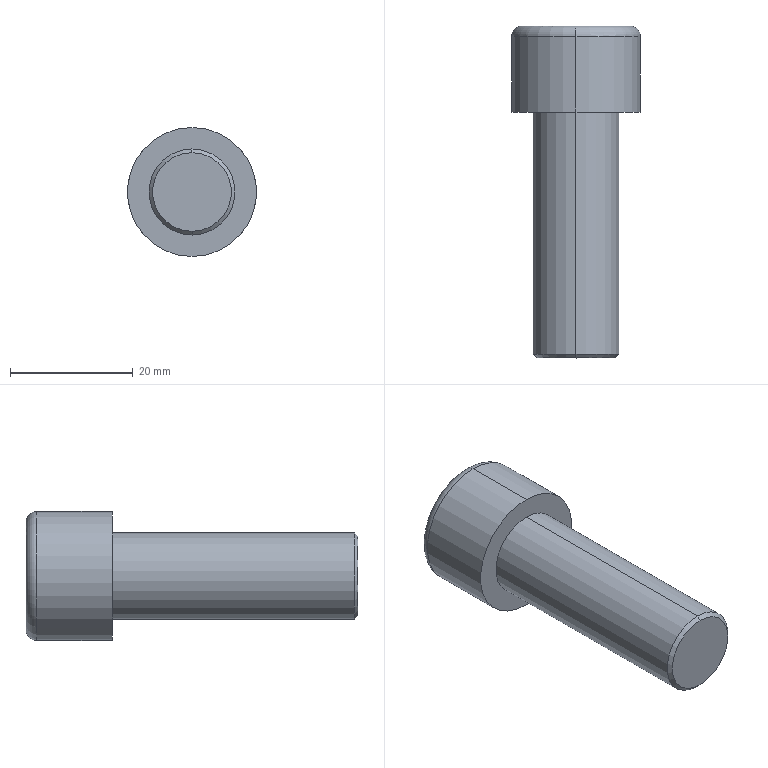Component | SolidWorks | hexagon socket head cap screws gb-100 | 1 solid | 25 faces | box 21 x 54 x 21 mm | volume 9954 mm3 | plane 15 | cone 4 | cylinder 4 | torus 2 | commonest cylinder face diameters 14 x2 21 x2
build123d program:
from build123d import *

# Parameters (mm, degrees)
SKETCH1_R           = 10.5
BASEHEAD_DEPTH      = 14
SKETCH2_R           = 7
BASEBODY_DEPTH      = 40
HEXAGONSOCKET_DEPTH = 7
TOPFILLET_R         = 1.75
CHAMFER1_SIZE       = 0.6


with BuildPart() as part:
    # Sketch1 → BaseHead (new body)
    with BuildSketch(Plane(origin=(0, 0, 0), x_dir=(0, 0, -1), z_dir=(1, 0, 0))):
        Circle(SKETCH1_R)
    extrude(amount=BASEHEAD_DEPTH)

    # Sketch2 → BaseBody (add)
    with BuildSketch(Plane(origin=(14, 0, 0), x_dir=(0, 0, -1), z_dir=(1, 0, 0))):
        Circle(SKETCH2_R)
    extrude(amount=BASEBODY_DEPTH)

    # Sketch3 → HexagonSocket (cut)
    with BuildSketch(Plane(origin=(0, 0, 0), x_dir=(0, 0, -1), z_dir=(1, 0, 0))):
        Polygon((6.928, 0), (3.464, 6), (-3.464, 6), (-6.928, 0), (-3.464, -6), (3.464, -6), align=None)
    extrude(amount=HEXAGONSOCKET_DEPTH, mode=Mode.SUBTRACT)

    # Sketch4 → Cut-Revolve1 (revolve, cut)
    with BuildSketch(Plane(origin=(-4.196, 0.75, 0), x_dir=(-1, 0, 0), z_dir=(0, 0, 1)), mode=Mode.PRIVATE) as cut_revolve1_sk:
        Polygon((-11.196, 6.75), (-14.66, 0.75), (-11.196, 0.75), align=None)
    revolve(cut_revolve1_sk.sketch.rotate(Axis((0.839, 0, 0), (-1, 0, 0)), 90), axis=Axis((0.839, 0, 0), (-1, 0, 0)), mode=Mode.SUBTRACT)

    # TopFillet
    topfillet_edges = [part.edges().sort_by_distance(p)[0] for p in [
        (0, 0, 10.5),
    ]]
    fillet(topfillet_edges, radius=TOPFILLET_R)

    # Chamfer1
    chamfer1_edges = [part.edges().sort_by_distance(p)[0] for p in [
        (54, 0, 7),
    ]]
    chamfer(chamfer1_edges, length=CHAMFER1_SIZE)


solid = part.part

# Placed as in the assembly
solid = solid.moved(Location((34.577, 214.019, 538.347), (0, 0, -90)))
STEP:
#1=COLOUR_RGB('',0.7922,0.8196,0.9333);
#2=FILL_AREA_STYLE_COLOUR('',#1);
#3=FILL_AREA_STYLE('',(#2));
#4=SURFACE_STYLE_FILL_AREA(#3);
#5=SURFACE_SIDE_STYLE('',(#4));
#6=SURFACE_STYLE_USAGE(.BOTH.,#5);
#7=PRESENTATION_STYLE_ASSIGNMENT((#6));
#8=CARTESIAN_POINT('',(1.361,6.3,21.447));
#9=VERTEX_POINT('',#8);
#10=CARTESIAN_POINT('',(1.361,6.3,20.943));
#11=VERTEX_POINT('',#10);
#12=CARTESIAN_POINT('',(1.361,6.3,21.195));
#13=DIRECTION('',(0.,-1.,0.));
#14=DIRECTION('',(-0.,0.,1.));
#15=AXIS2_PLACEMENT_3D('',#12,#13,#14);
#16=CIRCLE('',#15,0.252);
#17=EDGE_CURVE('',#9,#11,#16,.T.);
#18=ORIENTED_EDGE('',*,*,#17,.F.);
#19=CARTESIAN_POINT('',(1.361,6.324,21.47));
#20=VERTEX_POINT('',#19);
#21=CARTESIAN_POINT('',(1.361,6.3,21.447));
#22=DIRECTION('',(-0.,0.7071,0.7071));
#23=VECTOR('',#22,39.37);
#24=LINE('',#21,#23);
#25=EDGE_CURVE('',#9,#20,#24,.T.);
#26=ORIENTED_EDGE('',*,*,#25,.T.);
#27=CARTESIAN_POINT('',(1.361,6.324,20.919));
#28=VERTEX_POINT('',#27);
#29=CARTESIAN_POINT('',(1.361,6.324,21.195));
#30=DIRECTION('',(0.,1.,0.));
#31=DIRECTION('',(-0.,0.,1.));
#32=AXIS2_PLACEMENT_3D('',#29,#30,#31);
#33=CIRCLE('',#32,0.2756);
#34=EDGE_CURVE('',#28,#20,#33,.T.);
#35=ORIENTED_EDGE('',*,*,#34,.F.);
#36=CARTESIAN_POINT('',(1.361,6.3,20.943));
#37=DIRECTION('',(0.,0.7071,-0.7071));
#38=VECTOR('',#37,39.37);
#39=LINE('',#36,#38);
#40=EDGE_CURVE('',#11,#28,#39,.T.);
#41=ORIENTED_EDGE('',*,*,#40,.F.);
#42=EDGE_LOOP('',(#18,#26,#35,#41));
#43=FACE_OUTER_BOUND('',#42,.T.);
#44=CARTESIAN_POINT('',(1.361,6.3,21.195));
#45=DIRECTION('',(0.,1.,0.));
#46=DIRECTION('',(0.,0.,-1.));
#47=AXIS2_PLACEMENT_3D('',#44,#45,#46);
#48=CONICAL_SURFACE('',#47,0.252,0.7854);
#49=ADVANCED_FACE('',(#43),#48,.T.);
#50=CARTESIAN_POINT('',(1.361,8.426,20.85));
#51=VERTEX_POINT('',#50);
#52=CARTESIAN_POINT('',(1.361,8.426,21.539));
#53=VERTEX_POINT('',#52);
#54=CARTESIAN_POINT('',(1.361,8.426,21.195));
#55=DIRECTION('',(0.,1.,0.));
#56=DIRECTION('',(-0.,0.,1.));
#57=AXIS2_PLACEMENT_3D('',#54,#55,#56);
#58=CIRCLE('',#57,0.3445);
#59=EDGE_CURVE('',#51,#53,#58,.T.);
#60=ORIENTED_EDGE('',*,*,#59,.F.);
#61=CARTESIAN_POINT('',(1.361,8.357,20.781));
#62=VERTEX_POINT('',#61);
#63=CARTESIAN_POINT('',(1.361,8.357,20.85));
#64=DIRECTION('',(-1.,0.,-0.));
#65=DIRECTION('',(-0.,0.,1.));
#66=AXIS2_PLACEMENT_3D('',#63,#64,#65);
#67=CIRCLE('',#66,0.0689);
#68=EDGE_CURVE('',#51,#62,#67,.T.);
#69=ORIENTED_EDGE('',*,*,#68,.T.);
#70=CARTESIAN_POINT('',(1.361,8.357,21.608));
#71=VERTEX_POINT('',#70);
#72=CARTESIAN_POINT('',(1.361,8.357,21.195));
#73=DIRECTION('',(0.,-1.,0.));
#74=DIRECTION('',(-0.,0.,1.));
#75=AXIS2_PLACEMENT_3D('',#72,#73,#74);
#76=CIRCLE('',#75,0.4134);
#77=EDGE_CURVE('',#71,#62,#76,.T.);
#78=ORIENTED_EDGE('',*,*,#77,.F.);
#79=CARTESIAN_POINT('',(1.361,8.357,21.539));
#80=DIRECTION('',(1.,0.,0.));
#81=DIRECTION('',(0.,0.,-1.));
#82=AXIS2_PLACEMENT_3D('',#79,#80,#81);
#83=CIRCLE('',#82,0.0689);
#84=EDGE_CURVE('',#53,#71,#83,.T.);
#85=ORIENTED_EDGE('',*,*,#84,.F.);
#86=EDGE_LOOP('',(#60,#69,#78,#85));
#87=FACE_OUTER_BOUND('',#86,.T.);
#88=CARTESIAN_POINT('',(1.361,8.357,21.195));
#89=DIRECTION('',(0.,-1.,0.));
#90=DIRECTION('',(-0.,0.,1.));
#91=AXIS2_PLACEMENT_3D('',#88,#89,#90);
#92=TOROIDAL_SURFACE('',#91,0.3445,0.0689);
#93=ADVANCED_FACE('',(#87),#92,.T.);
#94=CARTESIAN_POINT('',(1.361,8.014,21.195));
#95=VERTEX_POINT('',#94);
#96=CARTESIAN_POINT('',(1.361,8.15,20.959));
#97=VERTEX_POINT('',#96);
#98=CARTESIAN_POINT('',(1.361,8.15,20.959));
#99=DIRECTION('',(0.,0.5,-0.866));
#100=VECTOR('',#99,39.37);
#101=LINE('',#98,#100);
#102=EDGE_CURVE('',#95,#97,#101,.T.);
#103=ORIENTED_EDGE('',*,*,#102,.F.);
#104=CARTESIAN_POINT('',(1.361,8.15,21.431));
#105=VERTEX_POINT('',#104);
#106=CARTESIAN_POINT('',(1.361,8.15,21.431));
#107=DIRECTION('',(-0.,0.5,0.866));
#108=VECTOR('',#107,39.37);
#109=LINE('',#106,#108);
#110=EDGE_CURVE('',#95,#105,#109,.T.);
#111=ORIENTED_EDGE('',*,*,#110,.T.);
#112=CARTESIAN_POINT('',(1.479,8.15,21.399));
#113=VERTEX_POINT('',#112);
#114=CARTESIAN_POINT('',(1.361,8.15,21.195));
#115=DIRECTION('',(0.,-1.,0.));
#116=DIRECTION('',(0.,0.,-1.));
#117=AXIS2_PLACEMENT_3D('',#114,#115,#116);
#118=CIRCLE('',#117,0.2362);
#119=EDGE_CURVE('',#113,#105,#118,.T.);
#120=ORIENTED_EDGE('',*,*,#119,.F.);
#121=CARTESIAN_POINT('',(1.598,8.15,21.195));
#122=VERTEX_POINT('',#121);
#123=CARTESIAN_POINT('',(1.361,8.15,21.195));
#124=DIRECTION('',(0.,-1.,0.));
#125=DIRECTION('',(0.,0.,-1.));
#126=AXIS2_PLACEMENT_3D('',#123,#124,#125);
#127=CIRCLE('',#126,0.2362);
#128=EDGE_CURVE('',#122,#113,#127,.T.);
#129=ORIENTED_EDGE('',*,*,#128,.F.);
#130=CARTESIAN_POINT('',(1.479,8.15,20.99));
#131=VERTEX_POINT('',#130);
#132=CARTESIAN_POINT('',(1.361,8.15,21.195));
#133=DIRECTION('',(0.,-1.,0.));
#134=DIRECTION('',(0.,0.,-1.));
#135=AXIS2_PLACEMENT_3D('',#132,#133,#134);
#136=CIRCLE('',#135,0.2362);
#137=EDGE_CURVE('',#131,#122,#136,.T.);
#138=ORIENTED_EDGE('',*,*,#137,.F.);
#139=CARTESIAN_POINT('',(1.361,8.15,21.195));
#140=DIRECTION('',(0.,-1.,0.));
#141=DIRECTION('',(0.,0.,-1.));
#142=AXIS2_PLACEMENT_3D('',#139,#140,#141);
#143=CIRCLE('',#142,0.2362);
#144=EDGE_CURVE('',#97,#131,#143,.T.);
#145=ORIENTED_EDGE('',*,*,#144,.F.);
#146=EDGE_LOOP('',(#103,#111,#120,#129,#138,#145));
#147=FACE_OUTER_BOUND('',#146,.T.);
#148=CARTESIAN_POINT('',(1.361,8.15,21.195));
#149=DIRECTION('',(0.,1.,0.));
#150=DIRECTION('',(0.,0.,-1.));
#151=AXIS2_PLACEMENT_3D('',#148,#149,#150);
#152=CONICAL_SURFACE('',#151,0.2362,1.047);
#153=ADVANCED_FACE('',(#147),#152,.F.);
#154=ORIENTED_EDGE('',*,*,#34,.T.);
#155=CARTESIAN_POINT('',(1.361,7.875,21.47));
#156=VERTEX_POINT('',#155);
#157=CARTESIAN_POINT('',(1.361,6.3,21.47));
#158=DIRECTION('',(0.,1.,0.));
#159=VECTOR('',#158,39.37);
#160=LINE('',#157,#159);
#161=EDGE_CURVE('',#20,#156,#160,.T.);
#162=ORIENTED_EDGE('',*,*,#161,.T.);
#163=CARTESIAN_POINT('',(1.361,7.875,20.919));
#164=VERTEX_POINT('',#163);
#165=CARTESIAN_POINT('',(1.361,7.875,21.195));
#166=DIRECTION('',(0.,-1.,0.));
#167=DIRECTION('',(-0.,0.,1.));
#168=AXIS2_PLACEMENT_3D('',#165,#166,#167);
#169=CIRCLE('',#168,0.2756);
#170=EDGE_CURVE('',#156,#164,#169,.T.);
#171=ORIENTED_EDGE('',*,*,#170,.T.);
#172=CARTESIAN_POINT('',(1.361,6.3,20.919));
#173=DIRECTION('',(0.,1.,0.));
#174=VECTOR('',#173,39.37);
#175=LINE('',#172,#174);
#176=EDGE_CURVE('',#28,#164,#175,.T.);
#177=ORIENTED_EDGE('',*,*,#176,.F.);
#178=EDGE_LOOP('',(#154,#162,#171,#177));
#179=FACE_OUTER_BOUND('',#178,.T.);
#180=CARTESIAN_POINT('',(1.361,6.3,21.195));
#181=DIRECTION('',(0.,1.,0.));
#182=DIRECTION('',(0.,0.,-1.));
#183=AXIS2_PLACEMENT_3D('',#180,#181,#182);
#184=CYLINDRICAL_SURFACE('',#183,0.2756);
#185=ADVANCED_FACE('',(#179),#184,.T.);
#186=CARTESIAN_POINT('',(1.361,7.875,21.608));
#187=VERTEX_POINT('',#186);
#188=CARTESIAN_POINT('',(1.361,7.875,20.781));
#189=VERTEX_POINT('',#188);
#190=CARTESIAN_POINT('',(1.361,7.875,21.195));
#191=DIRECTION('',(0.,-1.,0.));
#192=DIRECTION('',(-0.,0.,1.));
#193=AXIS2_PLACEMENT_3D('',#190,#191,#192);
#194=CIRCLE('',#193,0.4134);
#195=EDGE_CURVE('',#187,#189,#194,.T.);
#196=ORIENTED_EDGE('',*,*,#195,.F.);
#197=CARTESIAN_POINT('',(1.361,7.875,21.608));
#198=DIRECTION('',(0.,1.,0.));
#199=VECTOR('',#198,39.37);
#200=LINE('',#197,#199);
#201=EDGE_CURVE('',#187,#71,#200,.T.);
#202=ORIENTED_EDGE('',*,*,#201,.T.);
#203=ORIENTED_EDGE('',*,*,#77,.T.);
#204=CARTESIAN_POINT('',(1.361,7.875,20.781));
#205=DIRECTION('',(0.,1.,0.));
#206=VECTOR('',#205,39.37);
#207=LINE('',#204,#206);
#208=EDGE_CURVE('',#189,#62,#207,.T.);
#209=ORIENTED_EDGE('',*,*,#208,.F.);
#210=EDGE_LOOP('',(#196,#202,#203,#209));
#211=FACE_OUTER_BOUND('',#210,.T.);
#212=CARTESIAN_POINT('',(1.361,7.875,21.195));
#213=DIRECTION('',(0.,1.,0.));
#214=DIRECTION('',(0.,0.,-1.));
#215=AXIS2_PLACEMENT_3D('',#212,#213,#214);
#216=CYLINDRICAL_SURFACE('',#215,0.4134);
#217=ADVANCED_FACE('',(#211),#216,.T.);
#218=CARTESIAN_POINT('',(1.598,8.15,21.058));
#219=VERTEX_POINT('',#218);
#220=CARTESIAN_POINT('',(1.361,8.15,20.922));
#221=DIRECTION('',(0.866,0.,0.5));
#222=VECTOR('',#221,39.37);
#223=LINE('',#220,#222);
#224=EDGE_CURVE('',#131,#219,#223,.T.);
#225=ORIENTED_EDGE('',*,*,#224,.F.);
#226=ORIENTED_EDGE('',*,*,#137,.T.);
#227=CARTESIAN_POINT('',(1.598,8.15,21.058));
#228=DIRECTION('',(-0.,0.,1.));
#229=VECTOR('',#228,39.37);
#230=LINE('',#227,#229);
#231=EDGE_CURVE('',#219,#122,#230,.T.);
#232=ORIENTED_EDGE('',*,*,#231,.F.);
#233=EDGE_LOOP('',(#225,#226,#232));
#234=FACE_OUTER_BOUND('',#233,.T.);
#235=CARTESIAN_POINT('',(1.834,8.15,21.195));
#236=DIRECTION('',(0.,1.,0.));
#237=DIRECTION('',(0.,0.,-1.));
#238=AXIS2_PLACEMENT_3D('',#235,#236,#237);
#239=PLANE('',#238);
#240=ADVANCED_FACE('',(#234),#239,.T.);
#241=CARTESIAN_POINT('',(1.598,8.15,21.331));
#242=VERTEX_POINT('',#241);
#243=CARTESIAN_POINT('',(1.598,8.15,21.058));
#244=DIRECTION('',(-0.,0.,1.));
#245=VECTOR('',#244,39.37);
#246=LINE('',#243,#245);
#247=EDGE_CURVE('',#122,#242,#246,.T.);
#248=ORIENTED_EDGE('',*,*,#247,.F.);
#249=ORIENTED_EDGE('',*,*,#128,.T.);
#250=CARTESIAN_POINT('',(1.598,8.15,21.331));
#251=DIRECTION('',(-0.866,0.,0.5));
#252=VECTOR('',#251,39.37);
#253=LINE('',#250,#252);
#254=EDGE_CURVE('',#242,#113,#253,.T.);
#255=ORIENTED_EDGE('',*,*,#254,.F.);
#256=EDGE_LOOP('',(#248,#249,#255));
#257=FACE_OUTER_BOUND('',#256,.T.);
#258=CARTESIAN_POINT('',(1.834,8.15,21.195));
#259=DIRECTION('',(0.,1.,0.));
#260=DIRECTION('',(0.,0.,-1.));
#261=AXIS2_PLACEMENT_3D('',#258,#259,#260);
#262=PLANE('',#261);
#263=ADVANCED_FACE('',(#257),#262,.T.);
#264=CARTESIAN_POINT('',(1.361,8.15,21.468));
#265=VERTEX_POINT('',#264);
#266=CARTESIAN_POINT('',(1.598,8.15,21.331));
#267=DIRECTION('',(-0.866,0.,0.5));
#268=VECTOR('',#267,39.37);
#269=LINE('',#266,#268);
#270=EDGE_CURVE('',#113,#265,#269,.T.);
#271=ORIENTED_EDGE('',*,*,#270,.F.);
#272=ORIENTED_EDGE('',*,*,#119,.T.);
#273=CARTESIAN_POINT('',(1.243,8.15,21.399));
#274=VERTEX_POINT('',#273);
#275=CARTESIAN_POINT('',(1.361,8.15,21.195));
#276=DIRECTION('',(0.,-1.,0.));
#277=DIRECTION('',(-0.,0.,-1.));
#278=AXIS2_PLACEMENT_3D('',#275,#276,#277);
#279=CIRCLE('',#278,0.2362);
#280=EDGE_CURVE('',#105,#274,#279,.T.);
#281=ORIENTED_EDGE('',*,*,#280,.T.);
#282=CARTESIAN_POINT('',(1.361,8.15,21.468));
#283=DIRECTION('',(-0.866,0.,-0.5));
#284=VECTOR('',#283,39.37);
#285=LINE('',#282,#284);
#286=EDGE_CURVE('',#265,#274,#285,.T.);
#287=ORIENTED_EDGE('',*,*,#286,.F.);
#288=EDGE_LOOP('',(#271,#272,#281,#287));
#289=FACE_OUTER_BOUND('',#288,.T.);
#290=CARTESIAN_POINT('',(1.834,8.15,21.195));
#291=DIRECTION('',(0.,1.,0.));
#292=DIRECTION('',(0.,0.,-1.));
#293=AXIS2_PLACEMENT_3D('',#290,#291,#292);
#294=PLANE('',#293);
#295=ADVANCED_FACE('',(#289),#294,.T.);
#296=CARTESIAN_POINT('',(1.125,8.15,21.331));
#297=VERTEX_POINT('',#296);
#298=CARTESIAN_POINT('',(1.361,8.15,21.468));
#299=DIRECTION('',(-0.866,0.,-0.5));
#300=VECTOR('',#299,39.37);
#301=LINE('',#298,#300);
#302=EDGE_CURVE('',#274,#297,#301,.T.);
#303=ORIENTED_EDGE('',*,*,#302,.F.);
#304=CARTESIAN_POINT('',(1.125,8.15,21.195));
#305=VERTEX_POINT('',#304);
#306=CARTESIAN_POINT('',(1.361,8.15,21.195));
#307=DIRECTION('',(0.,-1.,0.));
#308=DIRECTION('',(-0.,0.,1.));
#309=AXIS2_PLACEMENT_3D('',#306,#307,#308);
#310=CIRCLE('',#309,0.2362);
#311=EDGE_CURVE('',#274,#305,#310,.T.);
#312=ORIENTED_EDGE('',*,*,#311,.T.);
#313=CARTESIAN_POINT('',(1.125,8.15,21.331));
#314=DIRECTION('',(0.,0.,-1.));
#315=VECTOR('',#314,39.37);
#316=LINE('',#313,#315);
#317=EDGE_CURVE('',#297,#305,#316,.T.);
#318=ORIENTED_EDGE('',*,*,#317,.F.);
#319=EDGE_LOOP('',(#303,#312,#318));
#320=FACE_OUTER_BOUND('',#319,.T.);
#321=CARTESIAN_POINT('',(1.834,8.15,21.195));
#322=DIRECTION('',(0.,1.,0.));
#323=DIRECTION('',(0.,0.,-1.));
#324=AXIS2_PLACEMENT_3D('',#321,#322,#323);
#325=PLANE('',#324);
#326=ADVANCED_FACE('',(#320),#325,.T.);
#327=CARTESIAN_POINT('',(1.125,8.15,21.058));
#328=VERTEX_POINT('',#327);
#329=CARTESIAN_POINT('',(1.125,8.15,21.331));
#330=DIRECTION('',(0.,0.,-1.));
#331=VECTOR('',#330,39.37);
#332=LINE('',#329,#331);
#333=EDGE_CURVE('',#305,#328,#332,.T.);
#334=ORIENTED_EDGE('',*,*,#333,.F.);
#335=CARTESIAN_POINT('',(1.243,8.15,20.99));
#336=VERTEX_POINT('',#335);
#337=CARTESIAN_POINT('',(1.361,8.15,21.195));
#338=DIRECTION('',(0.,-1.,0.));
#339=DIRECTION('',(0.,0.,-1.));
#340=AXIS2_PLACEMENT_3D('',#337,#338,#339);
#341=CIRCLE('',#340,0.2362);
#342=EDGE_CURVE('',#305,#336,#341,.T.);
#343=ORIENTED_EDGE('',*,*,#342,.T.);
#344=CARTESIAN_POINT('',(1.125,8.15,21.058));
#345=DIRECTION('',(0.866,0.,-0.5));
#346=VECTOR('',#345,39.37);
#347=LINE('',#344,#346);
#348=EDGE_CURVE('',#328,#336,#347,.T.);
#349=ORIENTED_EDGE('',*,*,#348,.F.);
#350=EDGE_LOOP('',(#334,#343,#349));
#351=FACE_OUTER_BOUND('',#350,.T.);
#352=CARTESIAN_POINT('',(1.834,8.15,21.195));
#353=DIRECTION('',(0.,1.,0.));
#354=DIRECTION('',(0.,0.,-1.));
#355=AXIS2_PLACEMENT_3D('',#352,#353,#354);
#356=PLANE('',#355);
#357=ADVANCED_FACE('',(#351),#356,.T.);
#358=CARTESIAN_POINT('',(1.361,8.15,20.922));
#359=VERTEX_POINT('',#358);
#360=CARTESIAN_POINT('',(1.125,8.15,21.058));
#361=DIRECTION('',(0.866,0.,-0.5));
#362=VECTOR('',#361,39.37);
#363=LINE('',#360,#362);
#364=EDGE_CURVE('',#336,#359,#363,.T.);
#365=ORIENTED_EDGE('',*,*,#364,.F.);
#366=CARTESIAN_POINT('',(1.361,8.15,21.195));
#367=DIRECTION('',(0.,-1.,0.));
#368=DIRECTION('',(-0.,0.,-1.));
#369=AXIS2_PLACEMENT_3D('',#366,#367,#368);
#370=CIRCLE('',#369,0.2362);
#371=EDGE_CURVE('',#336,#97,#370,.T.);
#372=ORIENTED_EDGE('',*,*,#371,.T.);
#373=ORIENTED_EDGE('',*,*,#144,.T.);
#374=CARTESIAN_POINT('',(1.361,8.15,20.922));
#375=DIRECTION('',(0.866,0.,0.5));
#376=VECTOR('',#375,39.37);
#377=LINE('',#374,#376);
#378=EDGE_CURVE('',#359,#131,#377,.T.);
#379=ORIENTED_EDGE('',*,*,#378,.F.);
#380=EDGE_LOOP('',(#365,#372,#373,#379));
#381=FACE_OUTER_BOUND('',#380,.T.);
#382=CARTESIAN_POINT('',(1.834,8.15,21.195));
#383=DIRECTION('',(0.,1.,0.));
#384=DIRECTION('',(0.,0.,-1.));
#385=AXIS2_PLACEMENT_3D('',#382,#383,#384);
#386=PLANE('',#385);
#387=ADVANCED_FACE('',(#381),#386,.T.);
#388=CARTESIAN_POINT('',(1.361,8.426,21.195));
#389=DIRECTION('',(0.,1.,0.));
#390=DIRECTION('',(-0.,0.,1.));
#391=AXIS2_PLACEMENT_3D('',#388,#389,#390);
#392=CIRCLE('',#391,0.3445);
#393=EDGE_CURVE('',#53,#51,#392,.T.);
#394=ORIENTED_EDGE('',*,*,#393,.T.);
#395=ORIENTED_EDGE('',*,*,#59,.T.);
#396=EDGE_LOOP('',(#394,#395));
#397=FACE_OUTER_BOUND('',#396,.T.);
#398=CARTESIAN_POINT('',(1.598,8.426,21.331));
#399=VERTEX_POINT('',#398);
#400=CARTESIAN_POINT('',(1.361,8.426,21.468));
#401=VERTEX_POINT('',#400);
#402=CARTESIAN_POINT('',(1.598,8.426,21.331));
#403=DIRECTION('',(-0.866,0.,0.5));
#404=VECTOR('',#403,39.37);
#405=LINE('',#402,#404);
#406=EDGE_CURVE('',#399,#401,#405,.T.);
#407=ORIENTED_EDGE('',*,*,#406,.T.);
#408=CARTESIAN_POINT('',(1.125,8.426,21.331));
#409=VERTEX_POINT('',#408);
#410=CARTESIAN_POINT('',(1.361,8.426,21.468));
#411=DIRECTION('',(-0.866,0.,-0.5));
#412=VECTOR('',#411,39.37);
#413=LINE('',#410,#412);
#414=EDGE_CURVE('',#401,#409,#413,.T.);
#415=ORIENTED_EDGE('',*,*,#414,.T.);
#416=CARTESIAN_POINT('',(1.125,8.426,21.058));
#417=VERTEX_POINT('',#416);
#418=CARTESIAN_POINT('',(1.125,8.426,21.331));
#419=DIRECTION('',(0.,0.,-1.));
#420=VECTOR('',#419,39.37);
#421=LINE('',#418,#420);
#422=EDGE_CURVE('',#409,#417,#421,.T.);
#423=ORIENTED_EDGE('',*,*,#422,.T.);
#424=CARTESIAN_POINT('',(1.361,8.426,20.922));
#425=VERTEX_POINT('',#424);
#426=CARTESIAN_POINT('',(1.125,8.426,21.058));
#427=DIRECTION('',(0.866,0.,-0.5));
#428=VECTOR('',#427,39.37);
#429=LINE('',#426,#428);
#430=EDGE_CURVE('',#417,#425,#429,.T.);
#431=ORIENTED_EDGE('',*,*,#430,.T.);
#432=CARTESIAN_POINT('',(1.598,8.426,21.058));
#433=VERTEX_POINT('',#432);
#434=CARTESIAN_POINT('',(1.361,8.426,20.922));
#435=DIRECTION('',(0.866,0.,0.5));
#436=VECTOR('',#435,39.37);
#437=LINE('',#434,#436);
#438=EDGE_CURVE('',#425,#433,#437,.T.);
#439=ORIENTED_EDGE('',*,*,#438,.T.);
#440=CARTESIAN_POINT('',(1.598,8.426,21.058));
#441=DIRECTION('',(-0.,0.,1.));
#442=VECTOR('',#441,39.37);
#443=LINE('',#440,#442);
#444=EDGE_CURVE('',#433,#399,#443,.T.);
#445=ORIENTED_EDGE('',*,*,#444,.T.);
#446=EDGE_LOOP('',(#407,#415,#423,#431,#439,#445));
#447=FACE_BOUND('',#446,.T.);
#448=CARTESIAN_POINT('',(1.361,8.426,21.195));
#449=DIRECTION('',(0.,-1.,0.));
#450=DIRECTION('',(-0.,0.,1.));
#451=AXIS2_PLACEMENT_3D('',#448,#449,#450);
#452=PLANE('',#451);
#453=ADVANCED_FACE('',(#397,#447),#452,.F.);
#454=CARTESIAN_POINT('',(1.361,7.875,21.195));
#455=DIRECTION('',(0.,-1.,0.));
#456=DIRECTION('',(-0.,0.,1.));
#457=AXIS2_PLACEMENT_3D('',#454,#455,#456);
#458=CIRCLE('',#457,0.4134);
#459=EDGE_CURVE('',#189,#187,#458,.T.);
#460=ORIENTED_EDGE('',*,*,#459,.T.);
#461=ORIENTED_EDGE('',*,*,#195,.T.);
#462=EDGE_LOOP('',(#460,#461));
#463=FACE_OUTER_BOUND('',#462,.T.);
#464=CARTESIAN_POINT('',(1.361,7.875,21.195));
#465=DIRECTION('',(0.,-1.,0.));
#466=DIRECTION('',(-0.,0.,1.));
#467=AXIS2_PLACEMENT_3D('',#464,#465,#466);
#468=CIRCLE('',#467,0.2756);
#469=EDGE_CURVE('',#164,#156,#468,.T.);
#470=ORIENTED_EDGE('',*,*,#469,.F.);
#471=ORIENTED_EDGE('',*,*,#170,.F.);
#472=EDGE_LOOP('',(#470,#471));
#473=FACE_BOUND('',#472,.T.);
#474=CARTESIAN_POINT('',(1.361,7.875,21.195));
#475=DIRECTION('',(0.,-1.,0.));
#476=DIRECTION('',(-0.,0.,1.));
#477=AXIS2_PLACEMENT_3D('',#474,#475,#476);
#478=PLANE('',#477);
#479=ADVANCED_FACE('',(#463,#473),#478,.T.);
#480=ORIENTED_EDGE('',*,*,#201,.F.);
#481=ORIENTED_EDGE('',*,*,#459,.F.);
#482=ORIENTED_EDGE('',*,*,#208,.T.);
#483=CARTESIAN_POINT('',(1.361,8.357,21.195));
#484=DIRECTION('',(0.,-1.,0.));
#485=DIRECTION('',(-0.,0.,1.));
#486=AXIS2_PLACEMENT_3D('',#483,#484,#485);
#487=CIRCLE('',#486,0.4134);
#488=EDGE_CURVE('',#62,#71,#487,.T.);
#489=ORIENTED_EDGE('',*,*,#488,.T.);
#490=EDGE_LOOP('',(#480,#481,#482,#489));
#491=FACE_OUTER_BOUND('',#490,.T.);
#492=CARTESIAN_POINT('',(1.361,7.875,21.195));
#493=DIRECTION('',(0.,1.,0.));
#494=DIRECTION('',(0.,0.,-1.));
#495=AXIS2_PLACEMENT_3D('',#492,#493,#494);
#496=CYLINDRICAL_SURFACE('',#495,0.4134);
#497=ADVANCED_FACE('',(#491),#496,.T.);
#498=ORIENTED_EDGE('',*,*,#161,.F.);
#499=CARTESIAN_POINT('',(1.361,6.324,21.195));
#500=DIRECTION('',(0.,1.,0.));
#501=DIRECTION('',(-0.,0.,1.));
#502=AXIS2_PLACEMENT_3D('',#499,#500,#501);
#503=CIRCLE('',#502,0.2756);
#504=EDGE_CURVE('',#20,#28,#503,.T.);
#505=ORIENTED_EDGE('',*,*,#504,.T.);
#506=ORIENTED_EDGE('',*,*,#176,.T.);
#507=ORIENTED_EDGE('',*,*,#469,.T.);
#508=EDGE_LOOP('',(#498,#505,#506,#507));
#509=FACE_OUTER_BOUND('',#508,.T.);
#510=CARTESIAN_POINT('',(1.361,6.3,21.195));
#511=DIRECTION('',(0.,1.,0.));
#512=DIRECTION('',(0.,0.,-1.));
#513=AXIS2_PLACEMENT_3D('',#510,#511,#512);
#514=CYLINDRICAL_SURFACE('',#513,0.2756);
#515=ADVANCED_FACE('',(#509),#514,.T.);
#516=CARTESIAN_POINT('',(1.361,6.3,21.195));
#517=DIRECTION('',(0.,-1.,0.));
#518=DIRECTION('',(-0.,0.,1.));
#519=AXIS2_PLACEMENT_3D('',#516,#517,#518);
#520=CIRCLE('',#519,0.252);
#521=EDGE_CURVE('',#11,#9,#520,.T.);
#522=ORIENTED_EDGE('',*,*,#521,.T.);
#523=ORIENTED_EDGE('',*,*,#17,.T.);
#524=EDGE_LOOP('',(#522,#523));
#525=FACE_OUTER_BOUND('',#524,.T.);
#526=CARTESIAN_POINT('',(1.361,6.3,21.195));
#527=DIRECTION('',(0.,-1.,0.));
#528=DIRECTION('',(-0.,0.,1.));
#529=AXIS2_PLACEMENT_3D('',#526,#527,#528);
#530=PLANE('',#529);
#531=ADVANCED_FACE('',(#525),#530,.T.);
#532=ORIENTED_EDGE('',*,*,#406,.F.);
#533=CARTESIAN_POINT('',(1.598,8.15,21.331));
#534=DIRECTION('',(0.,1.,0.));
#535=VECTOR('',#534,39.37);
#536=LINE('',#533,#535);
#537=EDGE_CURVE('',#242,#399,#536,.T.);
#538=ORIENTED_EDGE('',*,*,#537,.F.);
#539=ORIENTED_EDGE('',*,*,#254,.T.);
#540=ORIENTED_EDGE('',*,*,#270,.T.);
#541=CARTESIAN_POINT('',(1.361,8.15,21.468));
#542=DIRECTION('',(0.,1.,0.));
#543=VECTOR('',#542,39.37);
#544=LINE('',#541,#543);
#545=EDGE_CURVE('',#265,#401,#544,.T.);
#546=ORIENTED_EDGE('',*,*,#545,.T.);
#547=EDGE_LOOP('',(#532,#538,#539,#540,#546));
#548=FACE_OUTER_BOUND('',#547,.T.);
#549=CARTESIAN_POINT('',(1.598,8.15,21.331));
#550=DIRECTION('',(-0.5,0.,-0.866));
#551=DIRECTION('',(0.866,0.,-0.5));
#552=AXIS2_PLACEMENT_3D('',#549,#550,#551);
#553=PLANE('',#552);
#554=ADVANCED_FACE('',(#548),#553,.T.);
#555=ORIENTED_EDGE('',*,*,#414,.F.);
#556=ORIENTED_EDGE('',*,*,#545,.F.);
#557=ORIENTED_EDGE('',*,*,#286,.T.);
#558=ORIENTED_EDGE('',*,*,#302,.T.);
#559=CARTESIAN_POINT('',(1.125,8.15,21.331));
#560=DIRECTION('',(0.,1.,0.));
#561=VECTOR('',#560,39.37);
#562=LINE('',#559,#561);
#563=EDGE_CURVE('',#297,#409,#562,.T.);
#564=ORIENTED_EDGE('',*,*,#563,.T.);
#565=EDGE_LOOP('',(#555,#556,#557,#558,#564));
#566=FACE_OUTER_BOUND('',#565,.T.);
#567=CARTESIAN_POINT('',(1.361,8.15,21.468));
#568=DIRECTION('',(0.5,0.,-0.866));
#569=DIRECTION('',(0.866,0.,0.5));
#570=AXIS2_PLACEMENT_3D('',#567,#568,#569);
#571=PLANE('',#570);
#572=ADVANCED_FACE('',(#566),#571,.T.);
#573=ORIENTED_EDGE('',*,*,#422,.F.);
#574=ORIENTED_EDGE('',*,*,#563,.F.);
#575=ORIENTED_EDGE('',*,*,#317,.T.);
#576=ORIENTED_EDGE('',*,*,#333,.T.);
#577=CARTESIAN_POINT('',(1.125,8.15,21.058));
#578=DIRECTION('',(0.,1.,0.));
#579=VECTOR('',#578,39.37);
#580=LINE('',#577,#579);
#581=EDGE_CURVE('',#328,#417,#580,.T.);
#582=ORIENTED_EDGE('',*,*,#581,.T.);
#583=EDGE_LOOP('',(#573,#574,#575,#576,#582));
#584=FACE_OUTER_BOUND('',#583,.T.);
#585=CARTESIAN_POINT('',(1.125,8.15,21.331));
#586=DIRECTION('',(1.,0.,0.));
#587=DIRECTION('',(-0.,0.,1.));
#588=AXIS2_PLACEMENT_3D('',#585,#586,#587);
#589=PLANE('',#588);
#590=ADVANCED_FACE('',(#584),#589,.T.);
#591=ORIENTED_EDGE('',*,*,#430,.F.);
#592=ORIENTED_EDGE('',*,*,#581,.F.);
#593=ORIENTED_EDGE('',*,*,#348,.T.);
#594=ORIENTED_EDGE('',*,*,#364,.T.);
#595=CARTESIAN_POINT('',(1.361,8.15,20.922));
#596=DIRECTION('',(0.,1.,0.));
#597=VECTOR('',#596,39.37);
#598=LINE('',#595,#597);
#599=EDGE_CURVE('',#359,#425,#598,.T.);
#600=ORIENTED_EDGE('',*,*,#599,.T.);
#601=EDGE_LOOP('',(#591,#592,#593,#594,#600));
#602=FACE_OUTER_BOUND('',#601,.T.);
#603=CARTESIAN_POINT('',(1.125,8.15,21.058));
#604=DIRECTION('',(0.5,0.,0.866));
#605=DIRECTION('',(-0.866,0.,0.5));
#606=AXIS2_PLACEMENT_3D('',#603,#604,#605);
#607=PLANE('',#606);
#608=ADVANCED_FACE('',(#602),#607,.T.);
#609=ORIENTED_EDGE('',*,*,#438,.F.);
#610=ORIENTED_EDGE('',*,*,#599,.F.);
#611=ORIENTED_EDGE('',*,*,#378,.T.);
#612=ORIENTED_EDGE('',*,*,#224,.T.);
#613=CARTESIAN_POINT('',(1.598,8.15,21.058));
#614=DIRECTION('',(0.,1.,0.));
#615=VECTOR('',#614,39.37);
#616=LINE('',#613,#615);
#617=EDGE_CURVE('',#219,#433,#616,.T.);
#618=ORIENTED_EDGE('',*,*,#617,.T.);
#619=EDGE_LOOP('',(#609,#610,#611,#612,#618));
#620=FACE_OUTER_BOUND('',#619,.T.);
#621=CARTESIAN_POINT('',(1.361,8.15,20.922));
#622=DIRECTION('',(-0.5,0.,0.866));
#623=DIRECTION('',(-0.866,0.,-0.5));
#624=AXIS2_PLACEMENT_3D('',#621,#622,#623);
#625=PLANE('',#624);
#626=ADVANCED_FACE('',(#620),#625,.T.);
#627=ORIENTED_EDGE('',*,*,#444,.F.);
#628=ORIENTED_EDGE('',*,*,#617,.F.);
#629=ORIENTED_EDGE('',*,*,#231,.T.);
#630=ORIENTED_EDGE('',*,*,#247,.T.);
#631=ORIENTED_EDGE('',*,*,#537,.T.);
#632=EDGE_LOOP('',(#627,#628,#629,#630,#631));
#633=FACE_OUTER_BOUND('',#632,.T.);
#634=CARTESIAN_POINT('',(1.598,8.15,21.058));
#635=DIRECTION('',(-1.,0.,-0.));
#636=DIRECTION('',(0.,0.,-1.));
#637=AXIS2_PLACEMENT_3D('',#634,#635,#636);
#638=PLANE('',#637);
#639=ADVANCED_FACE('',(#633),#638,.T.);
#640=ORIENTED_EDGE('',*,*,#110,.F.);
#641=ORIENTED_EDGE('',*,*,#102,.T.);
#642=ORIENTED_EDGE('',*,*,#371,.F.);
#643=ORIENTED_EDGE('',*,*,#342,.F.);
#644=ORIENTED_EDGE('',*,*,#311,.F.);
#645=ORIENTED_EDGE('',*,*,#280,.F.);
#646=EDGE_LOOP('',(#640,#641,#642,#643,#644,#645));
#647=FACE_OUTER_BOUND('',#646,.T.);
#648=CARTESIAN_POINT('',(1.361,8.15,21.195));
#649=DIRECTION('',(0.,1.,0.));
#650=DIRECTION('',(0.,0.,-1.));
#651=AXIS2_PLACEMENT_3D('',#648,#649,#650);
#652=CONICAL_SURFACE('',#651,0.2362,1.047);
#653=ADVANCED_FACE('',(#647),#652,.F.);
#654=ORIENTED_EDGE('',*,*,#68,.F.);
#655=ORIENTED_EDGE('',*,*,#393,.F.);
#656=ORIENTED_EDGE('',*,*,#84,.T.);
#657=ORIENTED_EDGE('',*,*,#488,.F.);
#658=EDGE_LOOP('',(#654,#655,#656,#657));
#659=FACE_OUTER_BOUND('',#658,.T.);
#660=CARTESIAN_POINT('',(1.361,8.357,21.195));
#661=DIRECTION('',(0.,-1.,0.));
#662=DIRECTION('',(-0.,0.,1.));
#663=AXIS2_PLACEMENT_3D('',#660,#661,#662);
#664=TOROIDAL_SURFACE('',#663,0.3445,0.0689);
#665=ADVANCED_FACE('',(#659),#664,.T.);
#666=ORIENTED_EDGE('',*,*,#25,.F.);
#667=ORIENTED_EDGE('',*,*,#521,.F.);
#668=ORIENTED_EDGE('',*,*,#40,.T.);
#669=ORIENTED_EDGE('',*,*,#504,.F.);
#670=EDGE_LOOP('',(#666,#667,#668,#669));
#671=FACE_OUTER_BOUND('',#670,.T.);
#672=CARTESIAN_POINT('',(1.361,6.3,21.195));
#673=DIRECTION('',(0.,1.,0.));
#674=DIRECTION('',(0.,0.,-1.));
#675=AXIS2_PLACEMENT_3D('',#672,#673,#674);
#676=CONICAL_SURFACE('',#675,0.252,0.7854);
#677=ADVANCED_FACE('',(#671),#676,.T.);
#678=CLOSED_SHELL('',(#49,#93,#153,#185,#217,#240,#263,#295,#326,#357,#387,#453,#479,#497,#515,#531,#554,#572,#590,#608,#626,#639,#653,#665,#677));
#679=MANIFOLD_SOLID_BREP('',#678);
#680=STYLED_ITEM('',(#7),#679);
#681=PRESENTATION_LAYER_ASSIGNMENT('','',(#680));
#682=(LENGTH_UNIT()NAMED_UNIT(*)SI_UNIT($,.METRE.));
#683=LENGTH_MEASURE_WITH_UNIT(LENGTH_MEASURE(0.0254),#682);
#684=DIMENSIONAL_EXPONENTS(1.,0.,0.,0.,0.,0.,0.);
#685=(CONVERSION_BASED_UNIT('',#683)LENGTH_UNIT()NAMED_UNIT(#684));
#686=UNCERTAINTY_MEASURE_WITH_UNIT(LENGTH_MEASURE(0.00001),#685,'','');
#687=(NAMED_UNIT(*)PLANE_ANGLE_UNIT()SI_UNIT($,.RADIAN.));
#688=(NAMED_UNIT(*)SI_UNIT($,.STERADIAN.)SOLID_ANGLE_UNIT());
#689=(GEOMETRIC_REPRESENTATION_CONTEXT(3)GLOBAL_UNCERTAINTY_ASSIGNED_CONTEXT((#686))GLOBAL_UNIT_ASSIGNED_CONTEXT((#685,#687,#688))REPRESENTATION_CONTEXT('',''));
#690=MECHANICAL_DESIGN_GEOMETRIC_PRESENTATION_REPRESENTATION('',(#680),#689);
#691=CARTESIAN_POINT('',(0.,0.,0.));
#692=DIRECTION('',(0.,0.,1.));
#693=DIRECTION('',(1.,0.,0.));
#694=AXIS2_PLACEMENT_3D('',#691,#692,#693);
#695=(LENGTH_UNIT()NAMED_UNIT(*)SI_UNIT($,.METRE.));
#696=LENGTH_MEASURE_WITH_UNIT(LENGTH_MEASURE(0.0254),#695);
#697=DIMENSIONAL_EXPONENTS(1.,0.,0.,0.,0.,0.,0.);
#698=(CONVERSION_BASED_UNIT('',#696)LENGTH_UNIT()NAMED_UNIT(#697));
#699=UNCERTAINTY_MEASURE_WITH_UNIT(LENGTH_MEASURE(0.00001),#698,'','');
#700=(NAMED_UNIT(*)PLANE_ANGLE_UNIT()SI_UNIT($,.RADIAN.));
#701=(NAMED_UNIT(*)SI_UNIT($,.STERADIAN.)SOLID_ANGLE_UNIT());
#702=(GEOMETRIC_REPRESENTATION_CONTEXT(3)GLOBAL_UNCERTAINTY_ASSIGNED_CONTEXT((#699))GLOBAL_UNIT_ASSIGNED_CONTEXT((#698,#700,#701))REPRESENTATION_CONTEXT('',''));
#703=ADVANCED_BREP_SHAPE_REPRESENTATION('',(#679,#694),#702);